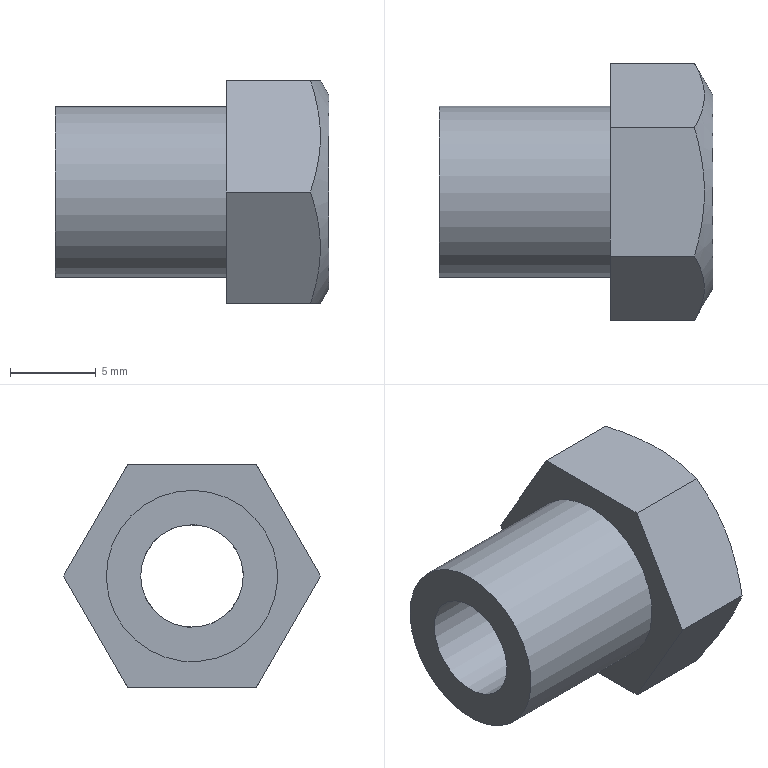Component | NX | PIPE_CAP_2 | 1 solid | 12 faces | box 16 x 15.01 x 13 mm | volume 1193 mm3 | plane 9 | cylinder 2 | cone 1 | commonest cylinder face diameters 10 x1 6 x1
STEP:
#1=CARTESIAN_POINT('',(0.,0.,0.));
#2=DIRECTION('',(0.,0.,1.));
#3=DIRECTION('',(1.,0.,0.));
#4=AXIS2_PLACEMENT_3D('',#1,#2,#3);
#5=CARTESIAN_POINT('',(-64.5,25.,18.5));
#6=VERTEX_POINT('',#5);
#7=CARTESIAN_POINT('',(-64.5,22.,18.5));
#8=DIRECTION('',(-1.,0.,0.));
#9=DIRECTION('',(0.,1.,0.));
#10=AXIS2_PLACEMENT_3D('',#7,#8,#9);
#11=CIRCLE('',#10,3.);
#12=CARTESIAN_POINT('',(-64.5,22.,18.5));
#13=DIRECTION('',(-1.,0.,0.));
#14=DIRECTION('',(0.,-0.5,0.866));
#15=AXIS2_PLACEMENT_3D('',#12,#13,#14);
#16=PLANE('',#15);
#17=CARTESIAN_POINT('',(0.,0.));
#18=DIRECTION('',(-0.5,0.866));
#19=AXIS2_PLACEMENT_2D('',#17,#18);
#20=CIRCLE('',#19,3.);
#21=(GEOMETRIC_REPRESENTATION_CONTEXT(2)PARAMETRIC_REPRESENTATION_CONTEXT()REPRESENTATION_CONTEXT('',''));
#22=DEFINITIONAL_REPRESENTATION('',(#20),#21);
#23=PCURVE('',#16,#22);
#24=CARTESIAN_POINT('',(-114.5,22.,18.5));
#25=DIRECTION('',(1.,0.,0.));
#26=DIRECTION('',(0.,0.5,-0.866));
#27=AXIS2_PLACEMENT_3D('',#24,#25,#26);
#28=CYLINDRICAL_SURFACE('',#27,3.);
#29=CARTESIAN_POINT('',(7.33,50.));
#30=DIRECTION('',(-1.,0.));
#31=VECTOR('',#30,1.);
#32=LINE('',#29,#31);
#33=(GEOMETRIC_REPRESENTATION_CONTEXT(2)PARAMETRIC_REPRESENTATION_CONTEXT()REPRESENTATION_CONTEXT('',''));
#34=DEFINITIONAL_REPRESENTATION('',(#32),#33);
#35=PCURVE('',#28,#34);
#36=SURFACE_CURVE('',#11,(#23,#35),.PCURVE_S1.);
#37=EDGE_CURVE('',#6,#6,#36,.T.);
#38=ORIENTED_EDGE('',*,*,#37,.T.);
#39=EDGE_LOOP('',(#38));
#40=FACE_BOUND('',#39,.T.);
#41=CARTESIAN_POINT('',(-64.5,19.185,23.375));
#42=VERTEX_POINT('',#41);
#43=CARTESIAN_POINT('',(-64.5,22.,18.5));
#44=DIRECTION('',(-1.,0.,0.));
#45=DIRECTION('',(0.,-0.5,0.866));
#46=AXIS2_PLACEMENT_3D('',#43,#44,#45);
#47=CIRCLE('',#46,5.629);
#48=CARTESIAN_POINT('',(0.,0.));
#49=DIRECTION('',(1.,0.));
#50=AXIS2_PLACEMENT_2D('',#48,#49);
#51=CIRCLE('',#50,5.629);
#52=(GEOMETRIC_REPRESENTATION_CONTEXT(2)PARAMETRIC_REPRESENTATION_CONTEXT()REPRESENTATION_CONTEXT('',''));
#53=DEFINITIONAL_REPRESENTATION('',(#51),#52);
#54=PCURVE('',#16,#53);
#55=CARTESIAN_POINT('',(-64.5,22.,18.5));
#56=DIRECTION('',(-1.,0.,0.));
#57=DIRECTION('',(0.,-0.5,0.866));
#58=AXIS2_PLACEMENT_3D('',#55,#56,#57);
#59=CONICAL_SURFACE('',#58,5.629,1.047);
#60=CARTESIAN_POINT('',(0.,0.));
#61=DIRECTION('',(1.,0.));
#62=VECTOR('',#61,1.);
#63=LINE('',#60,#62);
#64=(GEOMETRIC_REPRESENTATION_CONTEXT(2)PARAMETRIC_REPRESENTATION_CONTEXT()REPRESENTATION_CONTEXT('',''));
#65=DEFINITIONAL_REPRESENTATION('',(#63),#64);
#66=PCURVE('',#59,#65);
#67=SURFACE_CURVE('',#47,(#54,#66),.PCURVE_S1.);
#68=EDGE_CURVE('',#42,#42,#67,.T.);
#69=ORIENTED_EDGE('',*,*,#68,.F.);
#70=EDGE_LOOP('',(#69));
#71=FACE_BOUND('',#70,.T.);
#72=ADVANCED_FACE('',(#40,#71),#16,.F.);
#73=CARTESIAN_POINT('',(-80.5,20.5,21.098));
#74=VERTEX_POINT('',#73);
#75=CARTESIAN_POINT('',(-80.5,25.,18.5));
#76=VERTEX_POINT('',#75);
#77=CARTESIAN_POINT('',(-80.5,22.,18.5));
#78=DIRECTION('',(1.,0.,0.));
#79=DIRECTION('',(0.,-0.5,0.866));
#80=AXIS2_PLACEMENT_3D('',#77,#78,#79);
#81=CIRCLE('',#80,3.);
#82=CARTESIAN_POINT('',(-80.5,22.,18.5));
#83=DIRECTION('',(-1.,0.,0.));
#84=DIRECTION('',(0.,-0.5,0.866));
#85=AXIS2_PLACEMENT_3D('',#82,#83,#84);
#86=PLANE('',#85);
#87=CARTESIAN_POINT('',(3.,0.));
#88=CARTESIAN_POINT('',(3.,-5.196));
#89=CARTESIAN_POINT('',(-1.5,-2.598));
#90=CARTESIAN_POINT('',(-6.,-0.));
#91=CARTESIAN_POINT('',(-1.5,2.598));
#92=CARTESIAN_POINT('',(3.,5.196));
#93=CARTESIAN_POINT('',(3.,0.));
#94=(BOUNDED_CURVE()B_SPLINE_CURVE(2,(#87,#88,#89,#90,#91,#92,#93),.UNSPECIFIED.,.T.,.F.)B_SPLINE_CURVE_WITH_KNOTS((1,2,2,2,2,1),(-2.094,0.,2.094,4.189,6.283,8.378),.UNSPECIFIED.)CURVE()GEOMETRIC_REPRESENTATION_ITEM()RATIONAL_B_SPLINE_CURVE((1.,0.5,1.,0.5,1.,0.5,1.))REPRESENTATION_ITEM(''));
#95=(GEOMETRIC_REPRESENTATION_CONTEXT(2)PARAMETRIC_REPRESENTATION_CONTEXT()REPRESENTATION_CONTEXT('',''));
#96=DEFINITIONAL_REPRESENTATION('',(#94),#95);
#97=PCURVE('',#86,#96);
#98=CARTESIAN_POINT('',(3.142,34.));
#99=DIRECTION('',(1.,0.));
#100=VECTOR('',#99,1.);
#101=LINE('',#98,#100);
#102=(GEOMETRIC_REPRESENTATION_CONTEXT(2)PARAMETRIC_REPRESENTATION_CONTEXT()REPRESENTATION_CONTEXT('',''));
#103=DEFINITIONAL_REPRESENTATION('',(#101),#102);
#104=PCURVE('',#28,#103);
#105=SURFACE_CURVE('',#81,(#97,#104),.PCURVE_S1.);
#106=EDGE_CURVE('',#74,#76,#105,.T.);
#107=ORIENTED_EDGE('',*,*,#106,.T.);
#108=CARTESIAN_POINT('',(-80.5,22.,18.5));
#109=DIRECTION('',(1.,0.,0.));
#110=DIRECTION('',(0.,-0.5,0.866));
#111=AXIS2_PLACEMENT_3D('',#108,#109,#110);
#112=CIRCLE('',#111,3.);
#113=CARTESIAN_POINT('',(3.,0.));
#114=CARTESIAN_POINT('',(3.,-5.196));
#115=CARTESIAN_POINT('',(-1.5,-2.598));
#116=CARTESIAN_POINT('',(-6.,-0.));
#117=CARTESIAN_POINT('',(-1.5,2.598));
#118=CARTESIAN_POINT('',(3.,5.196));
#119=CARTESIAN_POINT('',(3.,0.));
#120=(BOUNDED_CURVE()B_SPLINE_CURVE(2,(#113,#114,#115,#116,#117,#118,#119),.UNSPECIFIED.,.T.,.F.)B_SPLINE_CURVE_WITH_KNOTS((1,2,2,2,2,1),(-2.094,0.,2.094,4.189,6.283,8.378),.UNSPECIFIED.)CURVE()GEOMETRIC_REPRESENTATION_ITEM()RATIONAL_B_SPLINE_CURVE((1.,0.5,1.,0.5,1.,0.5,1.))REPRESENTATION_ITEM(''));
#121=(GEOMETRIC_REPRESENTATION_CONTEXT(2)PARAMETRIC_REPRESENTATION_CONTEXT()REPRESENTATION_CONTEXT('',''));
#122=DEFINITIONAL_REPRESENTATION('',(#120),#121);
#123=PCURVE('',#86,#122);
#124=CARTESIAN_POINT('',(-3.142,34.));
#125=DIRECTION('',(1.,0.));
#126=VECTOR('',#125,1.);
#127=LINE('',#124,#126);
#128=(GEOMETRIC_REPRESENTATION_CONTEXT(2)PARAMETRIC_REPRESENTATION_CONTEXT()REPRESENTATION_CONTEXT('',''));
#129=DEFINITIONAL_REPRESENTATION('',(#127),#128);
#130=PCURVE('',#28,#129);
#131=SURFACE_CURVE('',#112,(#123,#130),.PCURVE_S1.);
#132=EDGE_CURVE('',#76,#74,#131,.T.);
#133=ORIENTED_EDGE('',*,*,#132,.T.);
#134=EDGE_LOOP('',(#107,#133));
#135=FACE_BOUND('',#134,.T.);
#136=CARTESIAN_POINT('',(-80.5,24.5,14.17));
#137=VERTEX_POINT('',#136);
#138=CARTESIAN_POINT('',(-80.5,22.,18.5));
#139=DIRECTION('',(1.,0.,0.));
#140=DIRECTION('',(0.,0.5,-0.866));
#141=AXIS2_PLACEMENT_3D('',#138,#139,#140);
#142=CIRCLE('',#141,5.);
#143=CARTESIAN_POINT('',(-5.,0.));
#144=CARTESIAN_POINT('',(-5.,8.66));
#145=CARTESIAN_POINT('',(2.5,4.33));
#146=CARTESIAN_POINT('',(10.,0.));
#147=CARTESIAN_POINT('',(2.5,-4.33));
#148=CARTESIAN_POINT('',(-5.,-8.66));
#149=CARTESIAN_POINT('',(-5.,0.));
#150=(BOUNDED_CURVE()B_SPLINE_CURVE(2,(#143,#144,#145,#146,#147,#148,#149),.UNSPECIFIED.,.T.,.F.)B_SPLINE_CURVE_WITH_KNOTS((1,2,2,2,2,1),(-2.094,0.,2.094,4.189,6.283,8.378),.UNSPECIFIED.)CURVE()GEOMETRIC_REPRESENTATION_ITEM()RATIONAL_B_SPLINE_CURVE((1.,0.5,1.,0.5,1.,0.5,1.))REPRESENTATION_ITEM(''));
#151=(GEOMETRIC_REPRESENTATION_CONTEXT(2)PARAMETRIC_REPRESENTATION_CONTEXT()REPRESENTATION_CONTEXT('',''));
#152=DEFINITIONAL_REPRESENTATION('',(#150),#151);
#153=PCURVE('',#86,#152);
#154=CARTESIAN_POINT('',(-80.5,22.,18.5));
#155=DIRECTION('',(1.,0.,0.));
#156=DIRECTION('',(0.,0.5,-0.866));
#157=AXIS2_PLACEMENT_3D('',#154,#155,#156);
#158=CYLINDRICAL_SURFACE('',#157,5.);
#159=CARTESIAN_POINT('',(0.,0.));
#160=DIRECTION('',(1.,0.));
#161=VECTOR('',#160,1.);
#162=LINE('',#159,#161);
#163=(GEOMETRIC_REPRESENTATION_CONTEXT(2)PARAMETRIC_REPRESENTATION_CONTEXT()REPRESENTATION_CONTEXT('',''));
#164=DEFINITIONAL_REPRESENTATION('',(#162),#163);
#165=PCURVE('',#158,#164);
#166=SURFACE_CURVE('',#142,(#153,#165),.PCURVE_S1.);
#167=EDGE_CURVE('',#137,#137,#166,.T.);
#168=ORIENTED_EDGE('',*,*,#167,.F.);
#169=EDGE_LOOP('',(#168));
#170=FACE_BOUND('',#169,.T.);
#171=ADVANCED_FACE('',(#135,#170),#86,.T.);
#172=CARTESIAN_POINT('',(-70.5,24.5,14.17));
#173=VERTEX_POINT('',#172);
#174=CARTESIAN_POINT('',(-70.5,22.,18.5));
#175=DIRECTION('',(-1.,0.,0.));
#176=DIRECTION('',(0.,0.5,-0.866));
#177=AXIS2_PLACEMENT_3D('',#174,#175,#176);
#178=CIRCLE('',#177,5.);
#179=CARTESIAN_POINT('',(6.283,10.));
#180=DIRECTION('',(-1.,0.));
#181=VECTOR('',#180,1.);
#182=LINE('',#179,#181);
#183=(GEOMETRIC_REPRESENTATION_CONTEXT(2)PARAMETRIC_REPRESENTATION_CONTEXT()REPRESENTATION_CONTEXT('',''));
#184=DEFINITIONAL_REPRESENTATION('',(#182),#183);
#185=PCURVE('',#158,#184);
#186=CARTESIAN_POINT('',(-70.5,22.,18.5));
#187=DIRECTION('',(-1.,0.,0.));
#188=DIRECTION('',(0.,-0.5,0.866));
#189=AXIS2_PLACEMENT_3D('',#186,#187,#188);
#190=PLANE('',#189);
#191=CARTESIAN_POINT('',(0.,0.));
#192=DIRECTION('',(-1.,0.));
#193=AXIS2_PLACEMENT_2D('',#191,#192);
#194=CIRCLE('',#193,5.);
#195=(GEOMETRIC_REPRESENTATION_CONTEXT(2)PARAMETRIC_REPRESENTATION_CONTEXT()REPRESENTATION_CONTEXT('',''));
#196=DEFINITIONAL_REPRESENTATION('',(#194),#195);
#197=PCURVE('',#190,#196);
#198=SURFACE_CURVE('',#178,(#185,#197),.PCURVE_S1.);
#199=EDGE_CURVE('',#173,#173,#198,.T.);
#200=ORIENTED_EDGE('',*,*,#199,.T.);
#201=CARTESIAN_POINT('',(-80.5,24.5,14.17));
#202=CARTESIAN_POINT('',(-70.5,24.5,14.17));
#203=B_SPLINE_CURVE_WITH_KNOTS('',1,(#201,#202),.UNSPECIFIED.,.F.,.F.,(2,2),(0.,10.),.PIECEWISE_BEZIER_KNOTS.);
#204=CARTESIAN_POINT('',(0.,0.));
#205=DIRECTION('',(0.,1.));
#206=VECTOR('',#205,1.);
#207=LINE('',#204,#206);
#208=(GEOMETRIC_REPRESENTATION_CONTEXT(2)PARAMETRIC_REPRESENTATION_CONTEXT()REPRESENTATION_CONTEXT('',''));
#209=DEFINITIONAL_REPRESENTATION('',(#207),#208);
#210=PCURVE('',#158,#209);
#211=CARTESIAN_POINT('',(6.283,0.));
#212=DIRECTION('',(0.,1.));
#213=VECTOR('',#212,1.);
#214=LINE('',#211,#213);
#215=(GEOMETRIC_REPRESENTATION_CONTEXT(2)PARAMETRIC_REPRESENTATION_CONTEXT()REPRESENTATION_CONTEXT('',''));
#216=DEFINITIONAL_REPRESENTATION('',(#214),#215);
#217=PCURVE('',#158,#216);
#218=SEAM_CURVE('',#203,(#210,#217),.PCURVE_S1.);
#219=EDGE_CURVE('',#137,#173,#218,.T.);
#220=ORIENTED_EDGE('',*,*,#219,.F.);
#221=ORIENTED_EDGE('',*,*,#167,.T.);
#222=ORIENTED_EDGE('',*,*,#219,.T.);
#223=EDGE_LOOP('',(#200,#220,#221,#222));
#224=FACE_BOUND('',#223,.T.);
#225=ADVANCED_FACE('',(#224),#158,.T.);
#226=CARTESIAN_POINT('',(-65.583,25.753,12.));
#227=VERTEX_POINT('',#226);
#228=CARTESIAN_POINT('',(-65.583,29.506,18.5));
#229=VERTEX_POINT('',#228);
#230=CARTESIAN_POINT('',(-65.583,25.753,12.));
#231=CARTESIAN_POINT('',(-65.23,26.366,13.061));
#232=CARTESIAN_POINT('',(-65.004,26.987,14.139));
#233=CARTESIAN_POINT('',(-65.002,28.264,16.349));
#234=CARTESIAN_POINT('',(-65.229,28.892,17.437));
#235=CARTESIAN_POINT('',(-65.583,29.506,18.5));
#236=B_SPLINE_CURVE_WITH_KNOTS('',3,(#230,#231,#232,#233,#234,#235),.UNSPECIFIED.,.F.,.F.,(4,2,4),(0.,0.5,1.),.UNSPECIFIED.);
#237=CARTESIAN_POINT('',(-64.5,29.506,18.5));
#238=DIRECTION('',(0.,0.866,-0.5));
#239=DIRECTION('',(0.,0.5,0.866));
#240=AXIS2_PLACEMENT_3D('',#237,#238,#239);
#241=PLANE('',#240);
#242=CARTESIAN_POINT('',(-7.506,-1.083));
#243=CARTESIAN_POINT('',(-6.28,-0.7296));
#244=CARTESIAN_POINT('',(-5.036,-0.5036));
#245=CARTESIAN_POINT('',(-2.484,-0.502));
#246=CARTESIAN_POINT('',(-1.227,-0.7291));
#247=CARTESIAN_POINT('',(0.,-1.083));
#248=B_SPLINE_CURVE_WITH_KNOTS('',3,(#242,#243,#244,#245,#246,#247),.UNSPECIFIED.,.F.,.F.,(4,2,4),(0.,0.5,1.),.UNSPECIFIED.);
#249=(GEOMETRIC_REPRESENTATION_CONTEXT(2)PARAMETRIC_REPRESENTATION_CONTEXT()REPRESENTATION_CONTEXT('',''));
#250=DEFINITIONAL_REPRESENTATION('',(#248),#249);
#251=PCURVE('',#241,#250);
#252=CARTESIAN_POINT('',(3.142,1.083));
#253=CARTESIAN_POINT('',(3.129,1.051));
#254=CARTESIAN_POINT('',(3.102,0.9889));
#255=CARTESIAN_POINT('',(3.061,0.9022));
#256=CARTESIAN_POINT('',(3.018,0.8227));
#257=CARTESIAN_POINT('',(2.973,0.7508));
#258=CARTESIAN_POINT('',(2.926,0.6871));
#259=CARTESIAN_POINT('',(2.878,0.632));
#260=CARTESIAN_POINT('',(2.828,0.586));
#261=CARTESIAN_POINT('',(2.777,0.5495));
#262=CARTESIAN_POINT('',(2.725,0.5229));
#263=CARTESIAN_POINT('',(2.673,0.5066));
#264=CARTESIAN_POINT('',(2.619,0.501));
#265=CARTESIAN_POINT('',(2.566,0.5062));
#266=CARTESIAN_POINT('',(2.513,0.5221));
#267=CARTESIAN_POINT('',(2.46,0.5484));
#268=CARTESIAN_POINT('',(2.409,0.5848));
#269=CARTESIAN_POINT('',(2.359,0.6308));
#270=CARTESIAN_POINT('',(2.311,0.686));
#271=CARTESIAN_POINT('',(2.264,0.7499));
#272=CARTESIAN_POINT('',(2.218,0.822));
#273=CARTESIAN_POINT('',(2.175,0.9018));
#274=CARTESIAN_POINT('',(2.134,0.9888));
#275=CARTESIAN_POINT('',(2.107,1.051));
#276=CARTESIAN_POINT('',(2.094,1.083));
#277=B_SPLINE_CURVE_WITH_KNOTS('',3,(#252,#253,#254,#255,#256,#257,#258,#259,#260,#261,#262,#263,#264,#265,#266,#267,#268,#269,#270,#271,#272,#273,#274,#275,#276),.UNSPECIFIED.,.F.,.F.,(4,1,1,1,1,1,1,1,1,1,1,1,1,1,1,1,1,1,1,1,1,1,4),(0.,0.04545,0.09091,0.1364,0.1818,0.2273,0.2727,0.3182,0.3636,0.4091,0.4545,0.5,0.5455,0.5909,0.6364,0.6818,0.7273,0.7727,0.8182,0.8636,0.9091,0.9545,1.),.QUASI_UNIFORM_KNOTS.);
#278=(GEOMETRIC_REPRESENTATION_CONTEXT(2)PARAMETRIC_REPRESENTATION_CONTEXT()REPRESENTATION_CONTEXT('',''));
#279=DEFINITIONAL_REPRESENTATION('',(#277),#278);
#280=PCURVE('',#59,#279);
#281=SURFACE_CURVE('',#236,(#251,#280),.PCURVE_S1.);
#282=EDGE_CURVE('',#227,#229,#281,.T.);
#283=ORIENTED_EDGE('',*,*,#282,.F.);
#284=CARTESIAN_POINT('',(-70.5,25.753,12.));
#285=VERTEX_POINT('',#284);
#286=CARTESIAN_POINT('',(-64.5,25.753,12.));
#287=DIRECTION('',(-1.,0.,0.));
#288=VECTOR('',#287,1.);
#289=LINE('',#286,#288);
#290=CARTESIAN_POINT('',(-7.506,0.));
#291=DIRECTION('',(0.,-1.));
#292=VECTOR('',#291,1.);
#293=LINE('',#290,#292);
#294=(GEOMETRIC_REPRESENTATION_CONTEXT(2)PARAMETRIC_REPRESENTATION_CONTEXT()REPRESENTATION_CONTEXT('',''));
#295=DEFINITIONAL_REPRESENTATION('',(#293),#294);
#296=PCURVE('',#241,#295);
#297=CARTESIAN_POINT('',(-64.5,25.753,12.));
#298=DIRECTION('',(0.,-0.,-1.));
#299=DIRECTION('',(0.,1.,-0.));
#300=AXIS2_PLACEMENT_3D('',#297,#298,#299);
#301=PLANE('',#300);
#302=CARTESIAN_POINT('',(0.,0.));
#303=DIRECTION('',(0.,-1.));
#304=VECTOR('',#303,1.);
#305=LINE('',#302,#304);
#306=(GEOMETRIC_REPRESENTATION_CONTEXT(2)PARAMETRIC_REPRESENTATION_CONTEXT()REPRESENTATION_CONTEXT('',''));
#307=DEFINITIONAL_REPRESENTATION('',(#305),#306);
#308=PCURVE('',#301,#307);
#309=SURFACE_CURVE('',#289,(#296,#308),.PCURVE_S1.);
#310=EDGE_CURVE('',#227,#285,#309,.T.);
#311=ORIENTED_EDGE('',*,*,#310,.T.);
#312=CARTESIAN_POINT('',(-70.5,29.506,18.5));
#313=VERTEX_POINT('',#312);
#314=CARTESIAN_POINT('',(-70.5,29.506,18.5));
#315=DIRECTION('',(0.,-0.5,-0.866));
#316=VECTOR('',#315,1.);
#317=LINE('',#314,#316);
#318=CARTESIAN_POINT('',(0.,-6.));
#319=DIRECTION('',(-1.,0.));
#320=VECTOR('',#319,1.);
#321=LINE('',#318,#320);
#322=(GEOMETRIC_REPRESENTATION_CONTEXT(2)PARAMETRIC_REPRESENTATION_CONTEXT()REPRESENTATION_CONTEXT('',''));
#323=DEFINITIONAL_REPRESENTATION('',(#321),#322);
#324=PCURVE('',#241,#323);
#325=CARTESIAN_POINT('',(-3.753,6.5));
#326=DIRECTION('',(-0.5,-0.866));
#327=VECTOR('',#326,1.);
#328=LINE('',#325,#327);
#329=(GEOMETRIC_REPRESENTATION_CONTEXT(2)PARAMETRIC_REPRESENTATION_CONTEXT()REPRESENTATION_CONTEXT('',''));
#330=DEFINITIONAL_REPRESENTATION('',(#328),#329);
#331=PCURVE('',#190,#330);
#332=SURFACE_CURVE('',#317,(#324,#331),.PCURVE_S1.);
#333=EDGE_CURVE('',#313,#285,#332,.T.);
#334=ORIENTED_EDGE('',*,*,#333,.F.);
#335=CARTESIAN_POINT('',(-64.5,29.506,18.5));
#336=DIRECTION('',(-1.,0.,0.));
#337=VECTOR('',#336,1.);
#338=LINE('',#335,#337);
#339=CARTESIAN_POINT('',(0.,0.));
#340=DIRECTION('',(0.,-1.));
#341=VECTOR('',#340,1.);
#342=LINE('',#339,#341);
#343=(GEOMETRIC_REPRESENTATION_CONTEXT(2)PARAMETRIC_REPRESENTATION_CONTEXT()REPRESENTATION_CONTEXT('',''));
#344=DEFINITIONAL_REPRESENTATION('',(#342),#343);
#345=PCURVE('',#241,#344);
#346=CARTESIAN_POINT('',(-64.5,25.753,25.));
#347=DIRECTION('',(0.,0.866,0.5));
#348=DIRECTION('',(0.,-0.5,0.866));
#349=AXIS2_PLACEMENT_3D('',#346,#347,#348);
#350=PLANE('',#349);
#351=CARTESIAN_POINT('',(-7.506,0.));
#352=DIRECTION('',(0.,-1.));
#353=VECTOR('',#352,1.);
#354=LINE('',#351,#353);
#355=(GEOMETRIC_REPRESENTATION_CONTEXT(2)PARAMETRIC_REPRESENTATION_CONTEXT()REPRESENTATION_CONTEXT('',''));
#356=DEFINITIONAL_REPRESENTATION('',(#354),#355);
#357=PCURVE('',#350,#356);
#358=SURFACE_CURVE('',#338,(#345,#357),.PCURVE_S1.);
#359=EDGE_CURVE('',#229,#313,#358,.T.);
#360=ORIENTED_EDGE('',*,*,#359,.F.);
#361=EDGE_LOOP('',(#283,#311,#334,#360));
#362=FACE_BOUND('',#361,.T.);
#363=ADVANCED_FACE('',(#362),#241,.T.);
#364=CARTESIAN_POINT('',(-65.583,18.247,12.));
#365=VERTEX_POINT('',#364);
#366=CARTESIAN_POINT('',(-65.583,18.247,12.));
#367=CARTESIAN_POINT('',(-65.23,19.473,12.));
#368=CARTESIAN_POINT('',(-65.004,20.717,12.));
#369=CARTESIAN_POINT('',(-65.002,23.269,12.));
#370=CARTESIAN_POINT('',(-65.229,24.526,12.));
#371=CARTESIAN_POINT('',(-65.583,25.753,12.));
#372=B_SPLINE_CURVE_WITH_KNOTS('',3,(#366,#367,#368,#369,#370,#371),.UNSPECIFIED.,.F.,.F.,(4,2,4),(0.,0.5,1.),.UNSPECIFIED.);
#373=CARTESIAN_POINT('',(-7.506,-1.083));
#374=CARTESIAN_POINT('',(-6.28,-0.7296));
#375=CARTESIAN_POINT('',(-5.036,-0.5036));
#376=CARTESIAN_POINT('',(-2.484,-0.502));
#377=CARTESIAN_POINT('',(-1.227,-0.7291));
#378=CARTESIAN_POINT('',(0.,-1.083));
#379=B_SPLINE_CURVE_WITH_KNOTS('',3,(#373,#374,#375,#376,#377,#378),.UNSPECIFIED.,.F.,.F.,(4,2,4),(0.,0.5,1.),.UNSPECIFIED.);
#380=(GEOMETRIC_REPRESENTATION_CONTEXT(2)PARAMETRIC_REPRESENTATION_CONTEXT()REPRESENTATION_CONTEXT('',''));
#381=DEFINITIONAL_REPRESENTATION('',(#379),#380);
#382=PCURVE('',#301,#381);
#383=CARTESIAN_POINT('',(4.189,1.083));
#384=CARTESIAN_POINT('',(4.176,1.051));
#385=CARTESIAN_POINT('',(4.15,0.9889));
#386=CARTESIAN_POINT('',(4.108,0.9022));
#387=CARTESIAN_POINT('',(4.065,0.8227));
#388=CARTESIAN_POINT('',(4.02,0.7508));
#389=CARTESIAN_POINT('',(3.974,0.6871));
#390=CARTESIAN_POINT('',(3.925,0.632));
#391=CARTESIAN_POINT('',(3.876,0.586));
#392=CARTESIAN_POINT('',(3.825,0.5495));
#393=CARTESIAN_POINT('',(3.773,0.5229));
#394=CARTESIAN_POINT('',(3.72,0.5066));
#395=CARTESIAN_POINT('',(3.666,0.501));
#396=CARTESIAN_POINT('',(3.613,0.5062));
#397=CARTESIAN_POINT('',(3.56,0.5221));
#398=CARTESIAN_POINT('',(3.507,0.5484));
#399=CARTESIAN_POINT('',(3.456,0.5848));
#400=CARTESIAN_POINT('',(3.406,0.6308));
#401=CARTESIAN_POINT('',(3.358,0.686));
#402=CARTESIAN_POINT('',(3.311,0.7499));
#403=CARTESIAN_POINT('',(3.266,0.822));
#404=CARTESIAN_POINT('',(3.222,0.9018));
#405=CARTESIAN_POINT('',(3.181,0.9888));
#406=CARTESIAN_POINT('',(3.154,1.051));
#407=CARTESIAN_POINT('',(3.142,1.083));
#408=B_SPLINE_CURVE_WITH_KNOTS('',3,(#383,#384,#385,#386,#387,#388,#389,#390,#391,#392,#393,#394,#395,#396,#397,#398,#399,#400,#401,#402,#403,#404,#405,#406,#407),.UNSPECIFIED.,.F.,.F.,(4,1,1,1,1,1,1,1,1,1,1,1,1,1,1,1,1,1,1,1,1,1,4),(0.,0.04545,0.09091,0.1364,0.1818,0.2273,0.2727,0.3182,0.3636,0.4091,0.4545,0.5,0.5455,0.5909,0.6364,0.6818,0.7273,0.7727,0.8182,0.8636,0.9091,0.9545,1.),.QUASI_UNIFORM_KNOTS.);
#409=(GEOMETRIC_REPRESENTATION_CONTEXT(2)PARAMETRIC_REPRESENTATION_CONTEXT()REPRESENTATION_CONTEXT('',''));
#410=DEFINITIONAL_REPRESENTATION('',(#408),#409);
#411=PCURVE('',#59,#410);
#412=SURFACE_CURVE('',#372,(#382,#411),.PCURVE_S1.);
#413=EDGE_CURVE('',#365,#227,#412,.T.);
#414=ORIENTED_EDGE('',*,*,#413,.F.);
#415=CARTESIAN_POINT('',(-70.5,18.247,12.));
#416=VERTEX_POINT('',#415);
#417=CARTESIAN_POINT('',(-64.5,18.247,12.));
#418=DIRECTION('',(-1.,0.,0.));
#419=VECTOR('',#418,1.);
#420=LINE('',#417,#419);
#421=CARTESIAN_POINT('',(-7.506,0.));
#422=DIRECTION('',(0.,-1.));
#423=VECTOR('',#422,1.);
#424=LINE('',#421,#423);
#425=(GEOMETRIC_REPRESENTATION_CONTEXT(2)PARAMETRIC_REPRESENTATION_CONTEXT()REPRESENTATION_CONTEXT('',''));
#426=DEFINITIONAL_REPRESENTATION('',(#424),#425);
#427=PCURVE('',#301,#426);
#428=CARTESIAN_POINT('',(-64.5,18.247,12.));
#429=DIRECTION('',(0.,-0.866,-0.5));
#430=DIRECTION('',(-1.,0.,0.));
#431=AXIS2_PLACEMENT_3D('',#428,#429,#430);
#432=PLANE('',#431);
#433=CARTESIAN_POINT('',(0.,0.));
#434=DIRECTION('',(1.,0.));
#435=VECTOR('',#434,1.);
#436=LINE('',#433,#435);
#437=(GEOMETRIC_REPRESENTATION_CONTEXT(2)PARAMETRIC_REPRESENTATION_CONTEXT()REPRESENTATION_CONTEXT('',''));
#438=DEFINITIONAL_REPRESENTATION('',(#436),#437);
#439=PCURVE('',#432,#438);
#440=SURFACE_CURVE('',#420,(#427,#439),.PCURVE_S1.);
#441=EDGE_CURVE('',#365,#416,#440,.T.);
#442=ORIENTED_EDGE('',*,*,#441,.T.);
#443=CARTESIAN_POINT('',(-70.5,25.753,12.));
#444=DIRECTION('',(0.,-1.,0.));
#445=VECTOR('',#444,1.);
#446=LINE('',#443,#445);
#447=CARTESIAN_POINT('',(0.,-6.));
#448=DIRECTION('',(-1.,0.));
#449=VECTOR('',#448,1.);
#450=LINE('',#447,#449);
#451=(GEOMETRIC_REPRESENTATION_CONTEXT(2)PARAMETRIC_REPRESENTATION_CONTEXT()REPRESENTATION_CONTEXT('',''));
#452=DEFINITIONAL_REPRESENTATION('',(#450),#451);
#453=PCURVE('',#301,#452);
#454=CARTESIAN_POINT('',(-7.506,0.));
#455=DIRECTION('',(0.5,-0.866));
#456=VECTOR('',#455,1.);
#457=LINE('',#454,#456);
#458=(GEOMETRIC_REPRESENTATION_CONTEXT(2)PARAMETRIC_REPRESENTATION_CONTEXT()REPRESENTATION_CONTEXT('',''));
#459=DEFINITIONAL_REPRESENTATION('',(#457),#458);
#460=PCURVE('',#190,#459);
#461=SURFACE_CURVE('',#446,(#453,#460),.PCURVE_S1.);
#462=EDGE_CURVE('',#285,#416,#461,.T.);
#463=ORIENTED_EDGE('',*,*,#462,.F.);
#464=ORIENTED_EDGE('',*,*,#310,.F.);
#465=EDGE_LOOP('',(#414,#442,#463,#464));
#466=FACE_BOUND('',#465,.T.);
#467=ADVANCED_FACE('',(#466),#301,.T.);
#468=CARTESIAN_POINT('',(-65.583,14.494,18.5));
#469=VERTEX_POINT('',#468);
#470=CARTESIAN_POINT('',(-65.583,14.494,18.5));
#471=CARTESIAN_POINT('',(-65.231,15.105,17.443));
#472=CARTESIAN_POINT('',(-65.003,15.737,16.347));
#473=CARTESIAN_POINT('',(-65.003,17.005,14.151));
#474=CARTESIAN_POINT('',(-65.233,17.641,13.051));
#475=CARTESIAN_POINT('',(-65.583,18.247,12.));
#476=B_SPLINE_CURVE_WITH_KNOTS('',3,(#470,#471,#472,#473,#474,#475),.UNSPECIFIED.,.F.,.F.,(4,2,4),(0.,0.5,1.),.UNSPECIFIED.);
#477=CARTESIAN_POINT('',(1.083,-7.506));
#478=CARTESIAN_POINT('',(0.731,-6.285));
#479=CARTESIAN_POINT('',(0.5027,-5.02));
#480=CARTESIAN_POINT('',(0.5029,-2.483));
#481=CARTESIAN_POINT('',(0.7331,-1.213));
#482=CARTESIAN_POINT('',(1.083,0.));
#483=B_SPLINE_CURVE_WITH_KNOTS('',3,(#477,#478,#479,#480,#481,#482),.UNSPECIFIED.,.F.,.F.,(4,2,4),(0.,0.5,1.),.UNSPECIFIED.);
#484=(GEOMETRIC_REPRESENTATION_CONTEXT(2)PARAMETRIC_REPRESENTATION_CONTEXT()REPRESENTATION_CONTEXT('',''));
#485=DEFINITIONAL_REPRESENTATION('',(#483),#484);
#486=PCURVE('',#432,#485);
#487=CARTESIAN_POINT('',(5.236,1.083));
#488=CARTESIAN_POINT('',(5.223,1.051));
#489=CARTESIAN_POINT('',(5.197,0.9892));
#490=CARTESIAN_POINT('',(5.156,0.9025));
#491=CARTESIAN_POINT('',(5.112,0.8227));
#492=CARTESIAN_POINT('',(5.067,0.7506));
#493=CARTESIAN_POINT('',(5.02,0.6866));
#494=CARTESIAN_POINT('',(4.972,0.6313));
#495=CARTESIAN_POINT('',(4.922,0.5852));
#496=CARTESIAN_POINT('',(4.87,0.5488));
#497=CARTESIAN_POINT('',(4.818,0.5224));
#498=CARTESIAN_POINT('',(4.765,0.5063));
#499=CARTESIAN_POINT('',(4.712,0.501));
#500=CARTESIAN_POINT('',(4.659,0.5064));
#501=CARTESIAN_POINT('',(4.606,0.5225));
#502=CARTESIAN_POINT('',(4.554,0.5491));
#503=CARTESIAN_POINT('',(4.503,0.5857));
#504=CARTESIAN_POINT('',(4.453,0.6319));
#505=CARTESIAN_POINT('',(4.404,0.6874));
#506=CARTESIAN_POINT('',(4.357,0.7514));
#507=CARTESIAN_POINT('',(4.312,0.8236));
#508=CARTESIAN_POINT('',(4.269,0.9032));
#509=CARTESIAN_POINT('',(4.228,0.9897));
#510=CARTESIAN_POINT('',(4.202,1.051));
#511=CARTESIAN_POINT('',(4.189,1.083));
#512=B_SPLINE_CURVE_WITH_KNOTS('',3,(#487,#488,#489,#490,#491,#492,#493,#494,#495,#496,#497,#498,#499,#500,#501,#502,#503,#504,#505,#506,#507,#508,#509,#510,#511),.UNSPECIFIED.,.F.,.F.,(4,1,1,1,1,1,1,1,1,1,1,1,1,1,1,1,1,1,1,1,1,1,4),(0.,0.04545,0.09091,0.1364,0.1818,0.2273,0.2727,0.3182,0.3636,0.4091,0.4545,0.5,0.5455,0.5909,0.6364,0.6818,0.7273,0.7727,0.8182,0.8636,0.9091,0.9545,1.),.QUASI_UNIFORM_KNOTS.);
#513=(GEOMETRIC_REPRESENTATION_CONTEXT(2)PARAMETRIC_REPRESENTATION_CONTEXT()REPRESENTATION_CONTEXT('',''));
#514=DEFINITIONAL_REPRESENTATION('',(#512),#513);
#515=PCURVE('',#59,#514);
#516=SURFACE_CURVE('',#476,(#486,#515),.PCURVE_S1.);
#517=EDGE_CURVE('',#469,#365,#516,.T.);
#518=ORIENTED_EDGE('',*,*,#517,.F.);
#519=CARTESIAN_POINT('',(-70.5,14.494,18.5));
#520=VERTEX_POINT('',#519);
#521=CARTESIAN_POINT('',(-64.5,14.494,18.5));
#522=DIRECTION('',(-1.,0.,0.));
#523=VECTOR('',#522,1.);
#524=LINE('',#521,#523);
#525=CARTESIAN_POINT('',(0.,-7.506));
#526=DIRECTION('',(1.,0.));
#527=VECTOR('',#526,1.);
#528=LINE('',#525,#527);
#529=(GEOMETRIC_REPRESENTATION_CONTEXT(2)PARAMETRIC_REPRESENTATION_CONTEXT()REPRESENTATION_CONTEXT('',''));
#530=DEFINITIONAL_REPRESENTATION('',(#528),#529);
#531=PCURVE('',#432,#530);
#532=CARTESIAN_POINT('',(-64.5,14.494,18.5));
#533=DIRECTION('',(0.,-0.866,0.5));
#534=DIRECTION('',(0.,-0.5,-0.866));
#535=AXIS2_PLACEMENT_3D('',#532,#533,#534);
#536=PLANE('',#535);
#537=CARTESIAN_POINT('',(0.,0.));
#538=DIRECTION('',(0.,-1.));
#539=VECTOR('',#538,1.);
#540=LINE('',#537,#539);
#541=(GEOMETRIC_REPRESENTATION_CONTEXT(2)PARAMETRIC_REPRESENTATION_CONTEXT()REPRESENTATION_CONTEXT('',''));
#542=DEFINITIONAL_REPRESENTATION('',(#540),#541);
#543=PCURVE('',#536,#542);
#544=SURFACE_CURVE('',#524,(#531,#543),.PCURVE_S1.);
#545=EDGE_CURVE('',#469,#520,#544,.T.);
#546=ORIENTED_EDGE('',*,*,#545,.T.);
#547=CARTESIAN_POINT('',(-70.5,18.247,12.));
#548=DIRECTION('',(0.,-0.5,0.866));
#549=VECTOR('',#548,1.);
#550=LINE('',#547,#549);
#551=CARTESIAN_POINT('',(6.,0.));
#552=DIRECTION('',(0.,-1.));
#553=VECTOR('',#552,1.);
#554=LINE('',#551,#553);
#555=(GEOMETRIC_REPRESENTATION_CONTEXT(2)PARAMETRIC_REPRESENTATION_CONTEXT()REPRESENTATION_CONTEXT('',''));
#556=DEFINITIONAL_REPRESENTATION('',(#554),#555);
#557=PCURVE('',#432,#556);
#558=CARTESIAN_POINT('',(-3.753,-6.5));
#559=DIRECTION('',(1.,0.));
#560=VECTOR('',#559,1.);
#561=LINE('',#558,#560);
#562=(GEOMETRIC_REPRESENTATION_CONTEXT(2)PARAMETRIC_REPRESENTATION_CONTEXT()REPRESENTATION_CONTEXT('',''));
#563=DEFINITIONAL_REPRESENTATION('',(#561),#562);
#564=PCURVE('',#190,#563);
#565=SURFACE_CURVE('',#550,(#557,#564),.PCURVE_S1.);
#566=EDGE_CURVE('',#416,#520,#565,.T.);
#567=ORIENTED_EDGE('',*,*,#566,.F.);
#568=ORIENTED_EDGE('',*,*,#441,.F.);
#569=EDGE_LOOP('',(#518,#546,#567,#568));
#570=FACE_BOUND('',#569,.T.);
#571=ADVANCED_FACE('',(#570),#432,.T.);
#572=CARTESIAN_POINT('',(-65.583,18.247,25.));
#573=VERTEX_POINT('',#572);
#574=CARTESIAN_POINT('',(-65.583,18.247,25.));
#575=CARTESIAN_POINT('',(-65.23,17.634,23.939));
#576=CARTESIAN_POINT('',(-65.004,17.013,22.861));
#577=CARTESIAN_POINT('',(-65.002,15.736,20.651));
#578=CARTESIAN_POINT('',(-65.229,15.108,19.563));
#579=CARTESIAN_POINT('',(-65.583,14.494,18.5));
#580=B_SPLINE_CURVE_WITH_KNOTS('',3,(#574,#575,#576,#577,#578,#579),.UNSPECIFIED.,.F.,.F.,(4,2,4),(0.,0.5,1.),.UNSPECIFIED.);
#581=CARTESIAN_POINT('',(-7.506,-1.083));
#582=CARTESIAN_POINT('',(-6.28,-0.7296));
#583=CARTESIAN_POINT('',(-5.036,-0.5036));
#584=CARTESIAN_POINT('',(-2.484,-0.502));
#585=CARTESIAN_POINT('',(-1.227,-0.7291));
#586=CARTESIAN_POINT('',(0.,-1.083));
#587=B_SPLINE_CURVE_WITH_KNOTS('',3,(#581,#582,#583,#584,#585,#586),.UNSPECIFIED.,.F.,.F.,(4,2,4),(0.,0.5,1.),.UNSPECIFIED.);
#588=(GEOMETRIC_REPRESENTATION_CONTEXT(2)PARAMETRIC_REPRESENTATION_CONTEXT()REPRESENTATION_CONTEXT('',''));
#589=DEFINITIONAL_REPRESENTATION('',(#587),#588);
#590=PCURVE('',#536,#589);
#591=CARTESIAN_POINT('',(6.283,1.083));
#592=CARTESIAN_POINT('',(6.27,1.051));
#593=CARTESIAN_POINT('',(6.244,0.9889));
#594=CARTESIAN_POINT('',(6.203,0.9022));
#595=CARTESIAN_POINT('',(6.16,0.8227));
#596=CARTESIAN_POINT('',(6.115,0.7508));
#597=CARTESIAN_POINT('',(6.068,0.6871));
#598=CARTESIAN_POINT('',(6.02,0.632));
#599=CARTESIAN_POINT('',(5.97,0.586));
#600=CARTESIAN_POINT('',(5.919,0.5495));
#601=CARTESIAN_POINT('',(5.867,0.5229));
#602=CARTESIAN_POINT('',(5.814,0.5066));
#603=CARTESIAN_POINT('',(5.761,0.501));
#604=CARTESIAN_POINT('',(5.707,0.5062));
#605=CARTESIAN_POINT('',(5.654,0.5221));
#606=CARTESIAN_POINT('',(5.602,0.5484));
#607=CARTESIAN_POINT('',(5.551,0.5848));
#608=CARTESIAN_POINT('',(5.501,0.6308));
#609=CARTESIAN_POINT('',(5.452,0.686));
#610=CARTESIAN_POINT('',(5.405,0.7499));
#611=CARTESIAN_POINT('',(5.36,0.822));
#612=CARTESIAN_POINT('',(5.317,0.9018));
#613=CARTESIAN_POINT('',(5.275,0.9888));
#614=CARTESIAN_POINT('',(5.249,1.051));
#615=CARTESIAN_POINT('',(5.236,1.083));
#616=B_SPLINE_CURVE_WITH_KNOTS('',3,(#591,#592,#593,#594,#595,#596,#597,#598,#599,#600,#601,#602,#603,#604,#605,#606,#607,#608,#609,#610,#611,#612,#613,#614,#615),.UNSPECIFIED.,.F.,.F.,(4,1,1,1,1,1,1,1,1,1,1,1,1,1,1,1,1,1,1,1,1,1,4),(0.,0.04545,0.09091,0.1364,0.1818,0.2273,0.2727,0.3182,0.3636,0.4091,0.4545,0.5,0.5455,0.5909,0.6364,0.6818,0.7273,0.7727,0.8182,0.8636,0.9091,0.9545,1.),.QUASI_UNIFORM_KNOTS.);
#617=(GEOMETRIC_REPRESENTATION_CONTEXT(2)PARAMETRIC_REPRESENTATION_CONTEXT()REPRESENTATION_CONTEXT('',''));
#618=DEFINITIONAL_REPRESENTATION('',(#616),#617);
#619=PCURVE('',#59,#618);
#620=SURFACE_CURVE('',#580,(#590,#619),.PCURVE_S1.);
#621=EDGE_CURVE('',#573,#469,#620,.T.);
#622=ORIENTED_EDGE('',*,*,#621,.F.);
#623=CARTESIAN_POINT('',(-70.5,18.247,25.));
#624=VERTEX_POINT('',#623);
#625=CARTESIAN_POINT('',(-64.5,18.247,25.));
#626=DIRECTION('',(-1.,0.,0.));
#627=VECTOR('',#626,1.);
#628=LINE('',#625,#627);
#629=CARTESIAN_POINT('',(-7.506,0.));
#630=DIRECTION('',(0.,-1.));
#631=VECTOR('',#630,1.);
#632=LINE('',#629,#631);
#633=(GEOMETRIC_REPRESENTATION_CONTEXT(2)PARAMETRIC_REPRESENTATION_CONTEXT()REPRESENTATION_CONTEXT('',''));
#634=DEFINITIONAL_REPRESENTATION('',(#632),#633);
#635=PCURVE('',#536,#634);
#636=CARTESIAN_POINT('',(-64.5,18.247,25.));
#637=DIRECTION('',(0.,0.,1.));
#638=DIRECTION('',(0.,-1.,0.));
#639=AXIS2_PLACEMENT_3D('',#636,#637,#638);
#640=PLANE('',#639);
#641=CARTESIAN_POINT('',(0.,0.));
#642=DIRECTION('',(0.,-1.));
#643=VECTOR('',#642,1.);
#644=LINE('',#641,#643);
#645=(GEOMETRIC_REPRESENTATION_CONTEXT(2)PARAMETRIC_REPRESENTATION_CONTEXT()REPRESENTATION_CONTEXT('',''));
#646=DEFINITIONAL_REPRESENTATION('',(#644),#645);
#647=PCURVE('',#640,#646);
#648=SURFACE_CURVE('',#628,(#635,#647),.PCURVE_S1.);
#649=EDGE_CURVE('',#573,#624,#648,.T.);
#650=ORIENTED_EDGE('',*,*,#649,.T.);
#651=CARTESIAN_POINT('',(-70.5,14.494,18.5));
#652=DIRECTION('',(0.,0.5,0.866));
#653=VECTOR('',#652,1.);
#654=LINE('',#651,#653);
#655=CARTESIAN_POINT('',(0.,-6.));
#656=DIRECTION('',(-1.,0.));
#657=VECTOR('',#656,1.);
#658=LINE('',#655,#657);
#659=(GEOMETRIC_REPRESENTATION_CONTEXT(2)PARAMETRIC_REPRESENTATION_CONTEXT()REPRESENTATION_CONTEXT('',''));
#660=DEFINITIONAL_REPRESENTATION('',(#658),#659);
#661=PCURVE('',#536,#660);
#662=CARTESIAN_POINT('',(3.753,-6.5));
#663=DIRECTION('',(0.5,0.866));
#664=VECTOR('',#663,1.);
#665=LINE('',#662,#664);
#666=(GEOMETRIC_REPRESENTATION_CONTEXT(2)PARAMETRIC_REPRESENTATION_CONTEXT()REPRESENTATION_CONTEXT('',''));
#667=DEFINITIONAL_REPRESENTATION('',(#665),#666);
#668=PCURVE('',#190,#667);
#669=SURFACE_CURVE('',#654,(#661,#668),.PCURVE_S1.);
#670=EDGE_CURVE('',#520,#624,#669,.T.);
#671=ORIENTED_EDGE('',*,*,#670,.F.);
#672=ORIENTED_EDGE('',*,*,#545,.F.);
#673=EDGE_LOOP('',(#622,#650,#671,#672));
#674=FACE_BOUND('',#673,.T.);
#675=ADVANCED_FACE('',(#674),#536,.T.);
#676=CARTESIAN_POINT('',(-65.583,25.753,25.));
#677=VERTEX_POINT('',#676);
#678=CARTESIAN_POINT('',(-65.583,25.753,25.));
#679=CARTESIAN_POINT('',(-65.23,24.527,25.));
#680=CARTESIAN_POINT('',(-65.004,23.283,25.));
#681=CARTESIAN_POINT('',(-65.002,20.731,25.));
#682=CARTESIAN_POINT('',(-65.229,19.474,25.));
#683=CARTESIAN_POINT('',(-65.583,18.247,25.));
#684=B_SPLINE_CURVE_WITH_KNOTS('',3,(#678,#679,#680,#681,#682,#683),.UNSPECIFIED.,.F.,.F.,(4,2,4),(0.,0.5,1.),.UNSPECIFIED.);
#685=CARTESIAN_POINT('',(-7.506,-1.083));
#686=CARTESIAN_POINT('',(-6.28,-0.7296));
#687=CARTESIAN_POINT('',(-5.036,-0.5036));
#688=CARTESIAN_POINT('',(-2.484,-0.502));
#689=CARTESIAN_POINT('',(-1.227,-0.7291));
#690=CARTESIAN_POINT('',(0.,-1.083));
#691=B_SPLINE_CURVE_WITH_KNOTS('',3,(#685,#686,#687,#688,#689,#690),.UNSPECIFIED.,.F.,.F.,(4,2,4),(0.,0.5,1.),.UNSPECIFIED.);
#692=(GEOMETRIC_REPRESENTATION_CONTEXT(2)PARAMETRIC_REPRESENTATION_CONTEXT()REPRESENTATION_CONTEXT('',''));
#693=DEFINITIONAL_REPRESENTATION('',(#691),#692);
#694=PCURVE('',#640,#693);
#695=CARTESIAN_POINT('',(1.047,1.083));
#696=CARTESIAN_POINT('',(1.034,1.051));
#697=CARTESIAN_POINT('',(1.008,0.9889));
#698=CARTESIAN_POINT('',(0.9667,0.9022));
#699=CARTESIAN_POINT('',(0.9236,0.8227));
#700=CARTESIAN_POINT('',(0.8787,0.7508));
#701=CARTESIAN_POINT('',(0.832,0.6871));
#702=CARTESIAN_POINT('',(0.7838,0.632));
#703=CARTESIAN_POINT('',(0.7341,0.586));
#704=CARTESIAN_POINT('',(0.6831,0.5495));
#705=CARTESIAN_POINT('',(0.631,0.5229));
#706=CARTESIAN_POINT('',(0.5782,0.5066));
#707=CARTESIAN_POINT('',(0.5247,0.501));
#708=CARTESIAN_POINT('',(0.4712,0.5062));
#709=CARTESIAN_POINT('',(0.4182,0.5221));
#710=CARTESIAN_POINT('',(0.3659,0.5484));
#711=CARTESIAN_POINT('',(0.3147,0.5848));
#712=CARTESIAN_POINT('',(0.2647,0.6308));
#713=CARTESIAN_POINT('',(0.2161,0.686));
#714=CARTESIAN_POINT('',(0.1692,0.7499));
#715=CARTESIAN_POINT('',(0.124,0.822));
#716=CARTESIAN_POINT('',(0.0807,0.9018));
#717=CARTESIAN_POINT('',(0.03925,0.9888));
#718=CARTESIAN_POINT('',(0.01287,1.051));
#719=CARTESIAN_POINT('',(0.,1.083));
#720=B_SPLINE_CURVE_WITH_KNOTS('',3,(#695,#696,#697,#698,#699,#700,#701,#702,#703,#704,#705,#706,#707,#708,#709,#710,#711,#712,#713,#714,#715,#716,#717,#718,#719),.UNSPECIFIED.,.F.,.F.,(4,1,1,1,1,1,1,1,1,1,1,1,1,1,1,1,1,1,1,1,1,1,4),(0.,0.04545,0.09091,0.1364,0.1818,0.2273,0.2727,0.3182,0.3636,0.4091,0.4545,0.5,0.5455,0.5909,0.6364,0.6818,0.7273,0.7727,0.8182,0.8636,0.9091,0.9545,1.),.QUASI_UNIFORM_KNOTS.);
#721=(GEOMETRIC_REPRESENTATION_CONTEXT(2)PARAMETRIC_REPRESENTATION_CONTEXT()REPRESENTATION_CONTEXT('',''));
#722=DEFINITIONAL_REPRESENTATION('',(#720),#721);
#723=PCURVE('',#59,#722);
#724=SURFACE_CURVE('',#684,(#694,#723),.PCURVE_S1.);
#725=EDGE_CURVE('',#677,#573,#724,.T.);
#726=ORIENTED_EDGE('',*,*,#725,.F.);
#727=CARTESIAN_POINT('',(-70.5,25.753,25.));
#728=VERTEX_POINT('',#727);
#729=CARTESIAN_POINT('',(-64.5,25.753,25.));
#730=DIRECTION('',(-1.,0.,0.));
#731=VECTOR('',#730,1.);
#732=LINE('',#729,#731);
#733=CARTESIAN_POINT('',(-7.506,0.));
#734=DIRECTION('',(0.,-1.));
#735=VECTOR('',#734,1.);
#736=LINE('',#733,#735);
#737=(GEOMETRIC_REPRESENTATION_CONTEXT(2)PARAMETRIC_REPRESENTATION_CONTEXT()REPRESENTATION_CONTEXT('',''));
#738=DEFINITIONAL_REPRESENTATION('',(#736),#737);
#739=PCURVE('',#640,#738);
#740=CARTESIAN_POINT('',(0.,0.));
#741=DIRECTION('',(0.,-1.));
#742=VECTOR('',#741,1.);
#743=LINE('',#740,#742);
#744=(GEOMETRIC_REPRESENTATION_CONTEXT(2)PARAMETRIC_REPRESENTATION_CONTEXT()REPRESENTATION_CONTEXT('',''));
#745=DEFINITIONAL_REPRESENTATION('',(#743),#744);
#746=PCURVE('',#350,#745);
#747=SURFACE_CURVE('',#732,(#739,#746),.PCURVE_S1.);
#748=EDGE_CURVE('',#677,#728,#747,.T.);
#749=ORIENTED_EDGE('',*,*,#748,.T.);
#750=CARTESIAN_POINT('',(-70.5,18.247,25.));
#751=DIRECTION('',(0.,1.,-0.));
#752=VECTOR('',#751,1.);
#753=LINE('',#750,#752);
#754=CARTESIAN_POINT('',(0.,-6.));
#755=DIRECTION('',(-1.,0.));
#756=VECTOR('',#755,1.);
#757=LINE('',#754,#756);
#758=(GEOMETRIC_REPRESENTATION_CONTEXT(2)PARAMETRIC_REPRESENTATION_CONTEXT()REPRESENTATION_CONTEXT('',''));
#759=DEFINITIONAL_REPRESENTATION('',(#757),#758);
#760=PCURVE('',#640,#759);
#761=CARTESIAN_POINT('',(7.506,0.));
#762=DIRECTION('',(-0.5,0.866));
#763=VECTOR('',#762,1.);
#764=LINE('',#761,#763);
#765=(GEOMETRIC_REPRESENTATION_CONTEXT(2)PARAMETRIC_REPRESENTATION_CONTEXT()REPRESENTATION_CONTEXT('',''));
#766=DEFINITIONAL_REPRESENTATION('',(#764),#765);
#767=PCURVE('',#190,#766);
#768=SURFACE_CURVE('',#753,(#760,#767),.PCURVE_S1.);
#769=EDGE_CURVE('',#624,#728,#768,.T.);
#770=ORIENTED_EDGE('',*,*,#769,.F.);
#771=ORIENTED_EDGE('',*,*,#649,.F.);
#772=EDGE_LOOP('',(#726,#749,#770,#771));
#773=FACE_BOUND('',#772,.T.);
#774=ADVANCED_FACE('',(#773),#640,.T.);
#775=CARTESIAN_POINT('',(-65.583,29.506,18.5));
#776=CARTESIAN_POINT('',(-65.233,28.899,19.551));
#777=CARTESIAN_POINT('',(-65.003,28.264,20.651));
#778=CARTESIAN_POINT('',(-65.003,26.996,22.847));
#779=CARTESIAN_POINT('',(-65.231,26.363,23.943));
#780=CARTESIAN_POINT('',(-65.583,25.753,25.));
#781=B_SPLINE_CURVE_WITH_KNOTS('',3,(#775,#776,#777,#778,#779,#780),.UNSPECIFIED.,.F.,.F.,(4,2,4),(0.,0.5,1.),.UNSPECIFIED.);
#782=CARTESIAN_POINT('',(-7.506,-1.083));
#783=CARTESIAN_POINT('',(-6.292,-0.7331));
#784=CARTESIAN_POINT('',(-5.022,-0.5029));
#785=CARTESIAN_POINT('',(-2.486,-0.5027));
#786=CARTESIAN_POINT('',(-1.221,-0.731));
#787=CARTESIAN_POINT('',(0.,-1.083));
#788=B_SPLINE_CURVE_WITH_KNOTS('',3,(#782,#783,#784,#785,#786,#787),.UNSPECIFIED.,.F.,.F.,(4,2,4),(0.,0.5,1.),.UNSPECIFIED.);
#789=(GEOMETRIC_REPRESENTATION_CONTEXT(2)PARAMETRIC_REPRESENTATION_CONTEXT()REPRESENTATION_CONTEXT('',''));
#790=DEFINITIONAL_REPRESENTATION('',(#788),#789);
#791=PCURVE('',#350,#790);
#792=CARTESIAN_POINT('',(2.094,1.083));
#793=CARTESIAN_POINT('',(2.082,1.051));
#794=CARTESIAN_POINT('',(2.056,0.9897));
#795=CARTESIAN_POINT('',(2.014,0.9032));
#796=CARTESIAN_POINT('',(1.971,0.8236));
#797=CARTESIAN_POINT('',(1.926,0.7514));
#798=CARTESIAN_POINT('',(1.879,0.6874));
#799=CARTESIAN_POINT('',(1.831,0.6319));
#800=CARTESIAN_POINT('',(1.781,0.5857));
#801=CARTESIAN_POINT('',(1.729,0.5491));
#802=CARTESIAN_POINT('',(1.677,0.5225));
#803=CARTESIAN_POINT('',(1.624,0.5064));
#804=CARTESIAN_POINT('',(1.571,0.501));
#805=CARTESIAN_POINT('',(1.518,0.5063));
#806=CARTESIAN_POINT('',(1.465,0.5224));
#807=CARTESIAN_POINT('',(1.413,0.5488));
#808=CARTESIAN_POINT('',(1.362,0.5852));
#809=CARTESIAN_POINT('',(1.312,0.6313));
#810=CARTESIAN_POINT('',(1.263,0.6866));
#811=CARTESIAN_POINT('',(1.216,0.7506));
#812=CARTESIAN_POINT('',(1.171,0.8227));
#813=CARTESIAN_POINT('',(1.128,0.9025));
#814=CARTESIAN_POINT('',(1.086,0.9892));
#815=CARTESIAN_POINT('',(1.06,1.051));
#816=CARTESIAN_POINT('',(1.047,1.083));
#817=B_SPLINE_CURVE_WITH_KNOTS('',3,(#792,#793,#794,#795,#796,#797,#798,#799,#800,#801,#802,#803,#804,#805,#806,#807,#808,#809,#810,#811,#812,#813,#814,#815,#816),.UNSPECIFIED.,.F.,.F.,(4,1,1,1,1,1,1,1,1,1,1,1,1,1,1,1,1,1,1,1,1,1,4),(0.,0.04545,0.09091,0.1364,0.1818,0.2273,0.2727,0.3182,0.3636,0.4091,0.4545,0.5,0.5455,0.5909,0.6364,0.6818,0.7273,0.7727,0.8182,0.8636,0.9091,0.9545,1.),.QUASI_UNIFORM_KNOTS.);
#818=(GEOMETRIC_REPRESENTATION_CONTEXT(2)PARAMETRIC_REPRESENTATION_CONTEXT()REPRESENTATION_CONTEXT('',''));
#819=DEFINITIONAL_REPRESENTATION('',(#817),#818);
#820=PCURVE('',#59,#819);
#821=SURFACE_CURVE('',#781,(#791,#820),.PCURVE_S1.);
#822=EDGE_CURVE('',#229,#677,#821,.T.);
#823=ORIENTED_EDGE('',*,*,#822,.F.);
#824=ORIENTED_EDGE('',*,*,#359,.T.);
#825=CARTESIAN_POINT('',(-70.5,25.753,25.));
#826=DIRECTION('',(0.,0.5,-0.866));
#827=VECTOR('',#826,1.);
#828=LINE('',#825,#827);
#829=CARTESIAN_POINT('',(0.,-6.));
#830=DIRECTION('',(-1.,0.));
#831=VECTOR('',#830,1.);
#832=LINE('',#829,#831);
#833=(GEOMETRIC_REPRESENTATION_CONTEXT(2)PARAMETRIC_REPRESENTATION_CONTEXT()REPRESENTATION_CONTEXT('',''));
#834=DEFINITIONAL_REPRESENTATION('',(#832),#833);
#835=PCURVE('',#350,#834);
#836=CARTESIAN_POINT('',(3.753,6.5));
#837=DIRECTION('',(-1.,0.));
#838=VECTOR('',#837,1.);
#839=LINE('',#836,#838);
#840=(GEOMETRIC_REPRESENTATION_CONTEXT(2)PARAMETRIC_REPRESENTATION_CONTEXT()REPRESENTATION_CONTEXT('',''));
#841=DEFINITIONAL_REPRESENTATION('',(#839),#840);
#842=PCURVE('',#190,#841);
#843=SURFACE_CURVE('',#828,(#835,#842),.PCURVE_S1.);
#844=EDGE_CURVE('',#728,#313,#843,.T.);
#845=ORIENTED_EDGE('',*,*,#844,.F.);
#846=ORIENTED_EDGE('',*,*,#748,.F.);
#847=EDGE_LOOP('',(#823,#824,#845,#846));
#848=FACE_BOUND('',#847,.T.);
#849=ADVANCED_FACE('',(#848),#350,.T.);
#850=ORIENTED_EDGE('',*,*,#199,.F.);
#851=EDGE_LOOP('',(#850));
#852=FACE_BOUND('',#851,.T.);
#853=ORIENTED_EDGE('',*,*,#333,.T.);
#854=ORIENTED_EDGE('',*,*,#462,.T.);
#855=ORIENTED_EDGE('',*,*,#566,.T.);
#856=ORIENTED_EDGE('',*,*,#670,.T.);
#857=ORIENTED_EDGE('',*,*,#769,.T.);
#858=ORIENTED_EDGE('',*,*,#844,.T.);
#859=EDGE_LOOP('',(#853,#854,#855,#856,#857,#858));
#860=FACE_BOUND('',#859,.T.);
#861=ADVANCED_FACE('',(#852,#860),#190,.T.);
#862=ORIENTED_EDGE('',*,*,#106,.T.);
#863=CARTESIAN_POINT('',(-80.5,25.,18.5));
#864=CARTESIAN_POINT('',(-64.5,25.,18.5));
#865=B_SPLINE_CURVE_WITH_KNOTS('',1,(#863,#864),.UNSPECIFIED.,.F.,.F.,(2,2),(34.,50.),.PIECEWISE_BEZIER_KNOTS.);
#866=CARTESIAN_POINT('',(7.33,0.));
#867=DIRECTION('',(0.,1.));
#868=VECTOR('',#867,1.);
#869=LINE('',#866,#868);
#870=(GEOMETRIC_REPRESENTATION_CONTEXT(2)PARAMETRIC_REPRESENTATION_CONTEXT()REPRESENTATION_CONTEXT('',''));
#871=DEFINITIONAL_REPRESENTATION('',(#869),#870);
#872=PCURVE('',#28,#871);
#873=CARTESIAN_POINT('',(1.047,0.));
#874=DIRECTION('',(0.,1.));
#875=VECTOR('',#874,1.);
#876=LINE('',#873,#875);
#877=(GEOMETRIC_REPRESENTATION_CONTEXT(2)PARAMETRIC_REPRESENTATION_CONTEXT()REPRESENTATION_CONTEXT('',''));
#878=DEFINITIONAL_REPRESENTATION('',(#876),#877);
#879=PCURVE('',#28,#878);
#880=SEAM_CURVE('',#865,(#872,#879),.PCURVE_S1.);
#881=EDGE_CURVE('',#76,#6,#880,.T.);
#882=ORIENTED_EDGE('',*,*,#881,.T.);
#883=ORIENTED_EDGE('',*,*,#37,.T.);
#884=ORIENTED_EDGE('',*,*,#881,.F.);
#885=ORIENTED_EDGE('',*,*,#132,.T.);
#886=EDGE_LOOP('',(#862,#882,#883,#884,#885));
#887=FACE_BOUND('',#886,.F.);
#888=ADVANCED_FACE('',(#887),#28,.F.);
#889=ORIENTED_EDGE('',*,*,#282,.T.);
#890=ORIENTED_EDGE('',*,*,#822,.T.);
#891=ORIENTED_EDGE('',*,*,#725,.T.);
#892=CARTESIAN_POINT('',(-64.5,19.185,23.375));
#893=CARTESIAN_POINT('',(-65.583,18.247,25.));
#894=B_SPLINE_CURVE_WITH_KNOTS('',1,(#892,#893),.UNSPECIFIED.,.F.,.F.,(2,2),(0.,2.167),.PIECEWISE_BEZIER_KNOTS.);
#895=CARTESIAN_POINT('',(0.,0.));
#896=DIRECTION('',(0.,1.));
#897=VECTOR('',#896,1.);
#898=LINE('',#895,#897);
#899=(GEOMETRIC_REPRESENTATION_CONTEXT(2)PARAMETRIC_REPRESENTATION_CONTEXT()REPRESENTATION_CONTEXT('',''));
#900=DEFINITIONAL_REPRESENTATION('',(#898),#899);
#901=PCURVE('',#59,#900);
#902=CARTESIAN_POINT('',(6.283,0.));
#903=DIRECTION('',(0.,1.));
#904=VECTOR('',#903,1.);
#905=LINE('',#902,#904);
#906=(GEOMETRIC_REPRESENTATION_CONTEXT(2)PARAMETRIC_REPRESENTATION_CONTEXT()REPRESENTATION_CONTEXT('',''));
#907=DEFINITIONAL_REPRESENTATION('',(#905),#906);
#908=PCURVE('',#59,#907);
#909=SEAM_CURVE('',#894,(#901,#908),.PCURVE_S1.);
#910=EDGE_CURVE('',#42,#573,#909,.T.);
#911=ORIENTED_EDGE('',*,*,#910,.F.);
#912=ORIENTED_EDGE('',*,*,#68,.T.);
#913=ORIENTED_EDGE('',*,*,#910,.T.);
#914=ORIENTED_EDGE('',*,*,#621,.T.);
#915=ORIENTED_EDGE('',*,*,#517,.T.);
#916=ORIENTED_EDGE('',*,*,#413,.T.);
#917=EDGE_LOOP('',(#889,#890,#891,#911,#912,#913,#914,#915,#916));
#918=FACE_BOUND('',#917,.T.);
#919=ADVANCED_FACE('',(#918),#59,.T.);
#920=CLOSED_SHELL('',(#72,#171,#225,#363,#467,#571,#675,#774,#849,#861,#888,#919));
#921=MANIFOLD_SOLID_BREP('',#920);
#922=(LENGTH_UNIT()NAMED_UNIT(*)SI_UNIT(.MILLI.,.METRE.));
#923=UNCERTAINTY_MEASURE_WITH_UNIT(LENGTH_MEASURE(0.0005),#922,'','');
#924=(NAMED_UNIT(*)PLANE_ANGLE_UNIT()SI_UNIT($,.RADIAN.));
#925=(NAMED_UNIT(*)SI_UNIT($,.STERADIAN.)SOLID_ANGLE_UNIT());
#926=(GEOMETRIC_REPRESENTATION_CONTEXT(3)GLOBAL_UNCERTAINTY_ASSIGNED_CONTEXT((#923))GLOBAL_UNIT_ASSIGNED_CONTEXT((#922,#924,#925))REPRESENTATION_CONTEXT('',''));
#927=ADVANCED_BREP_SHAPE_REPRESENTATION('',(#4,#921),#926);